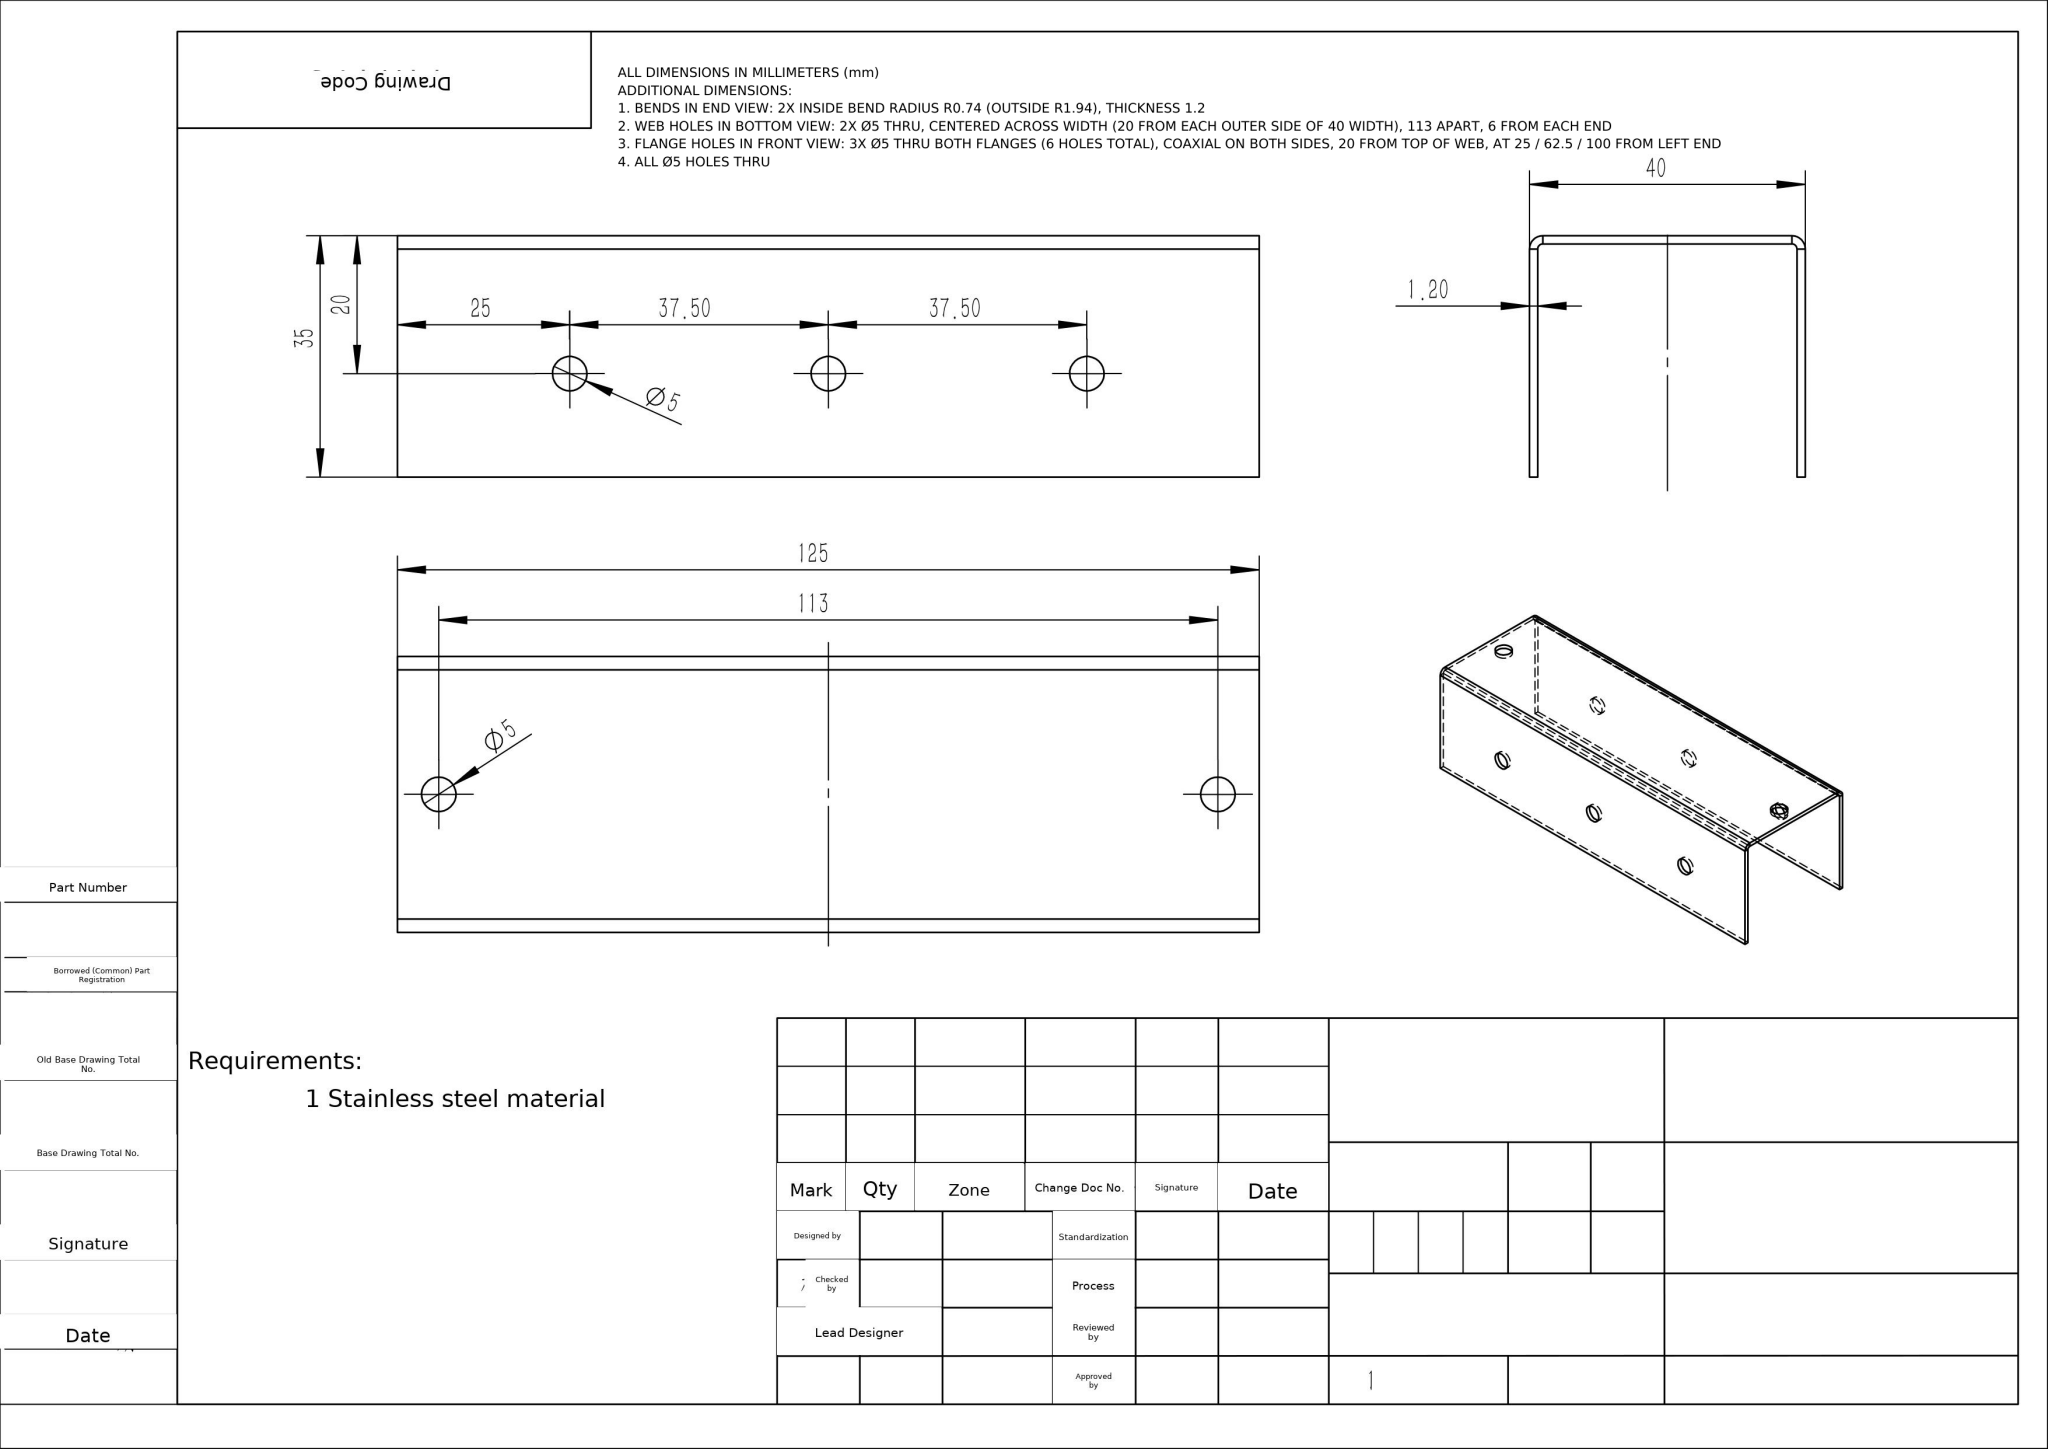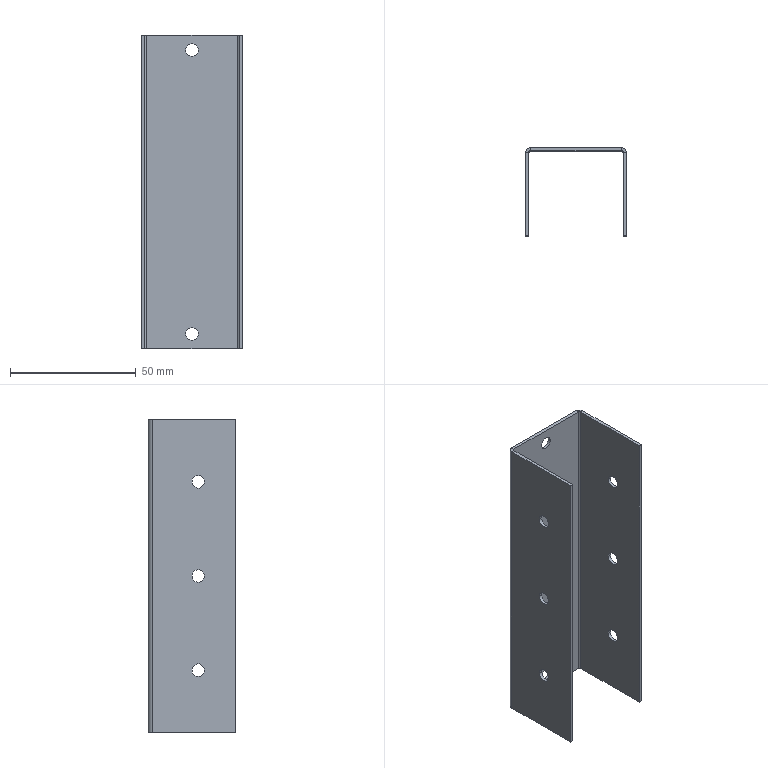Part | NX | mm | 1 solid | 38 faces | box 40 x 35 x 125 mm | volume 15779 mm3 | cylinder 20 | plane 18 | commonest cylinder face diameters 5 x16 1.473 x2 3.873 x2